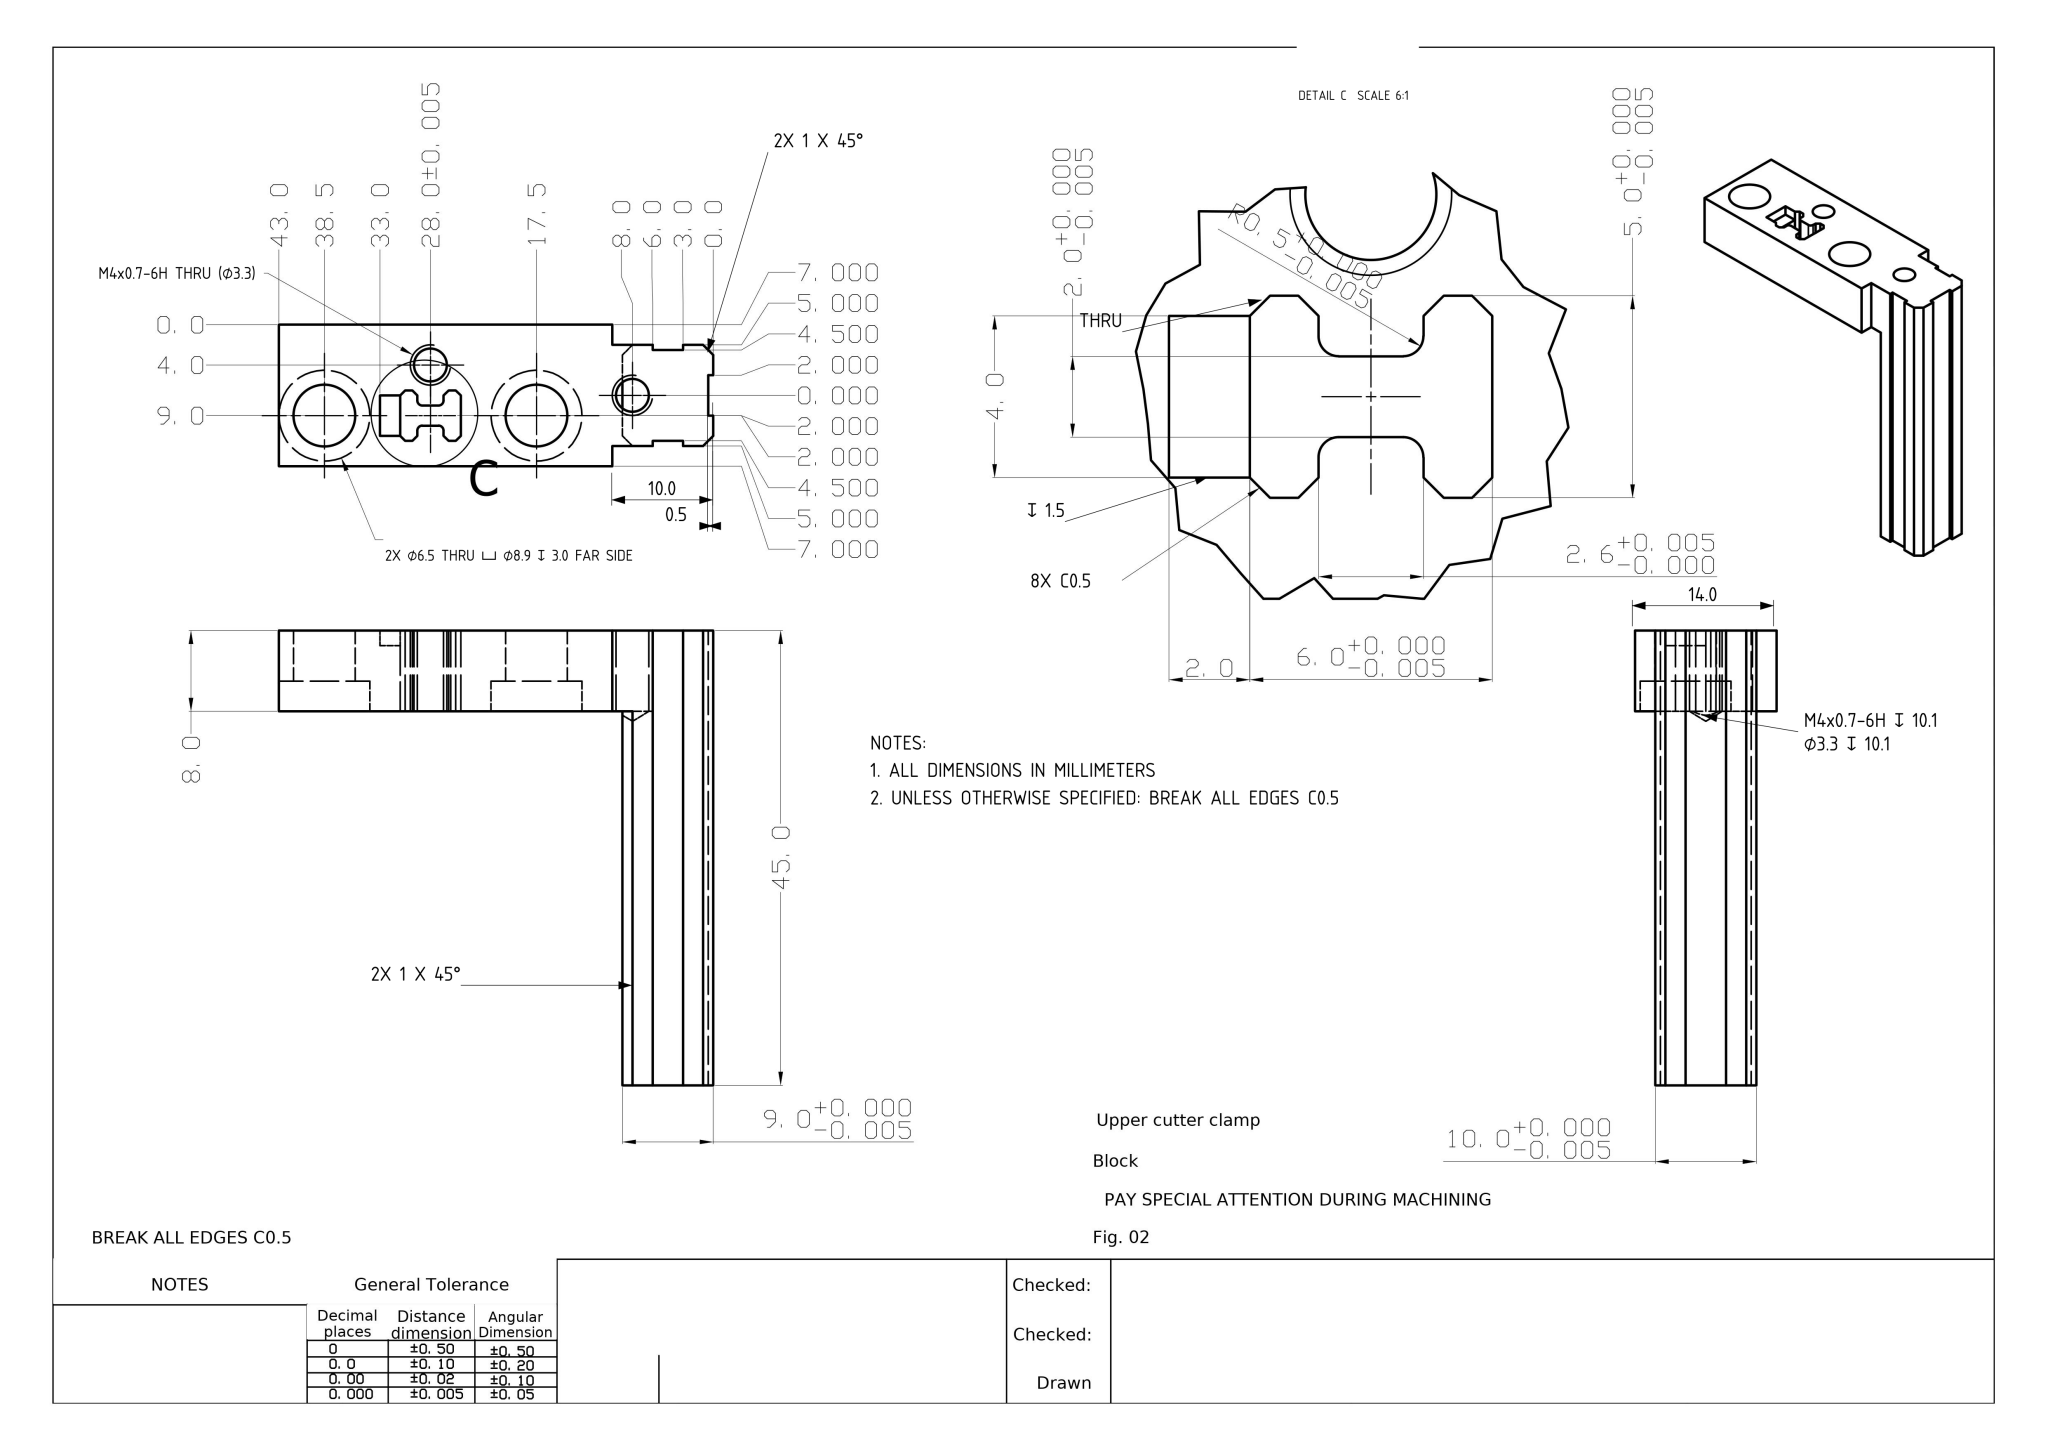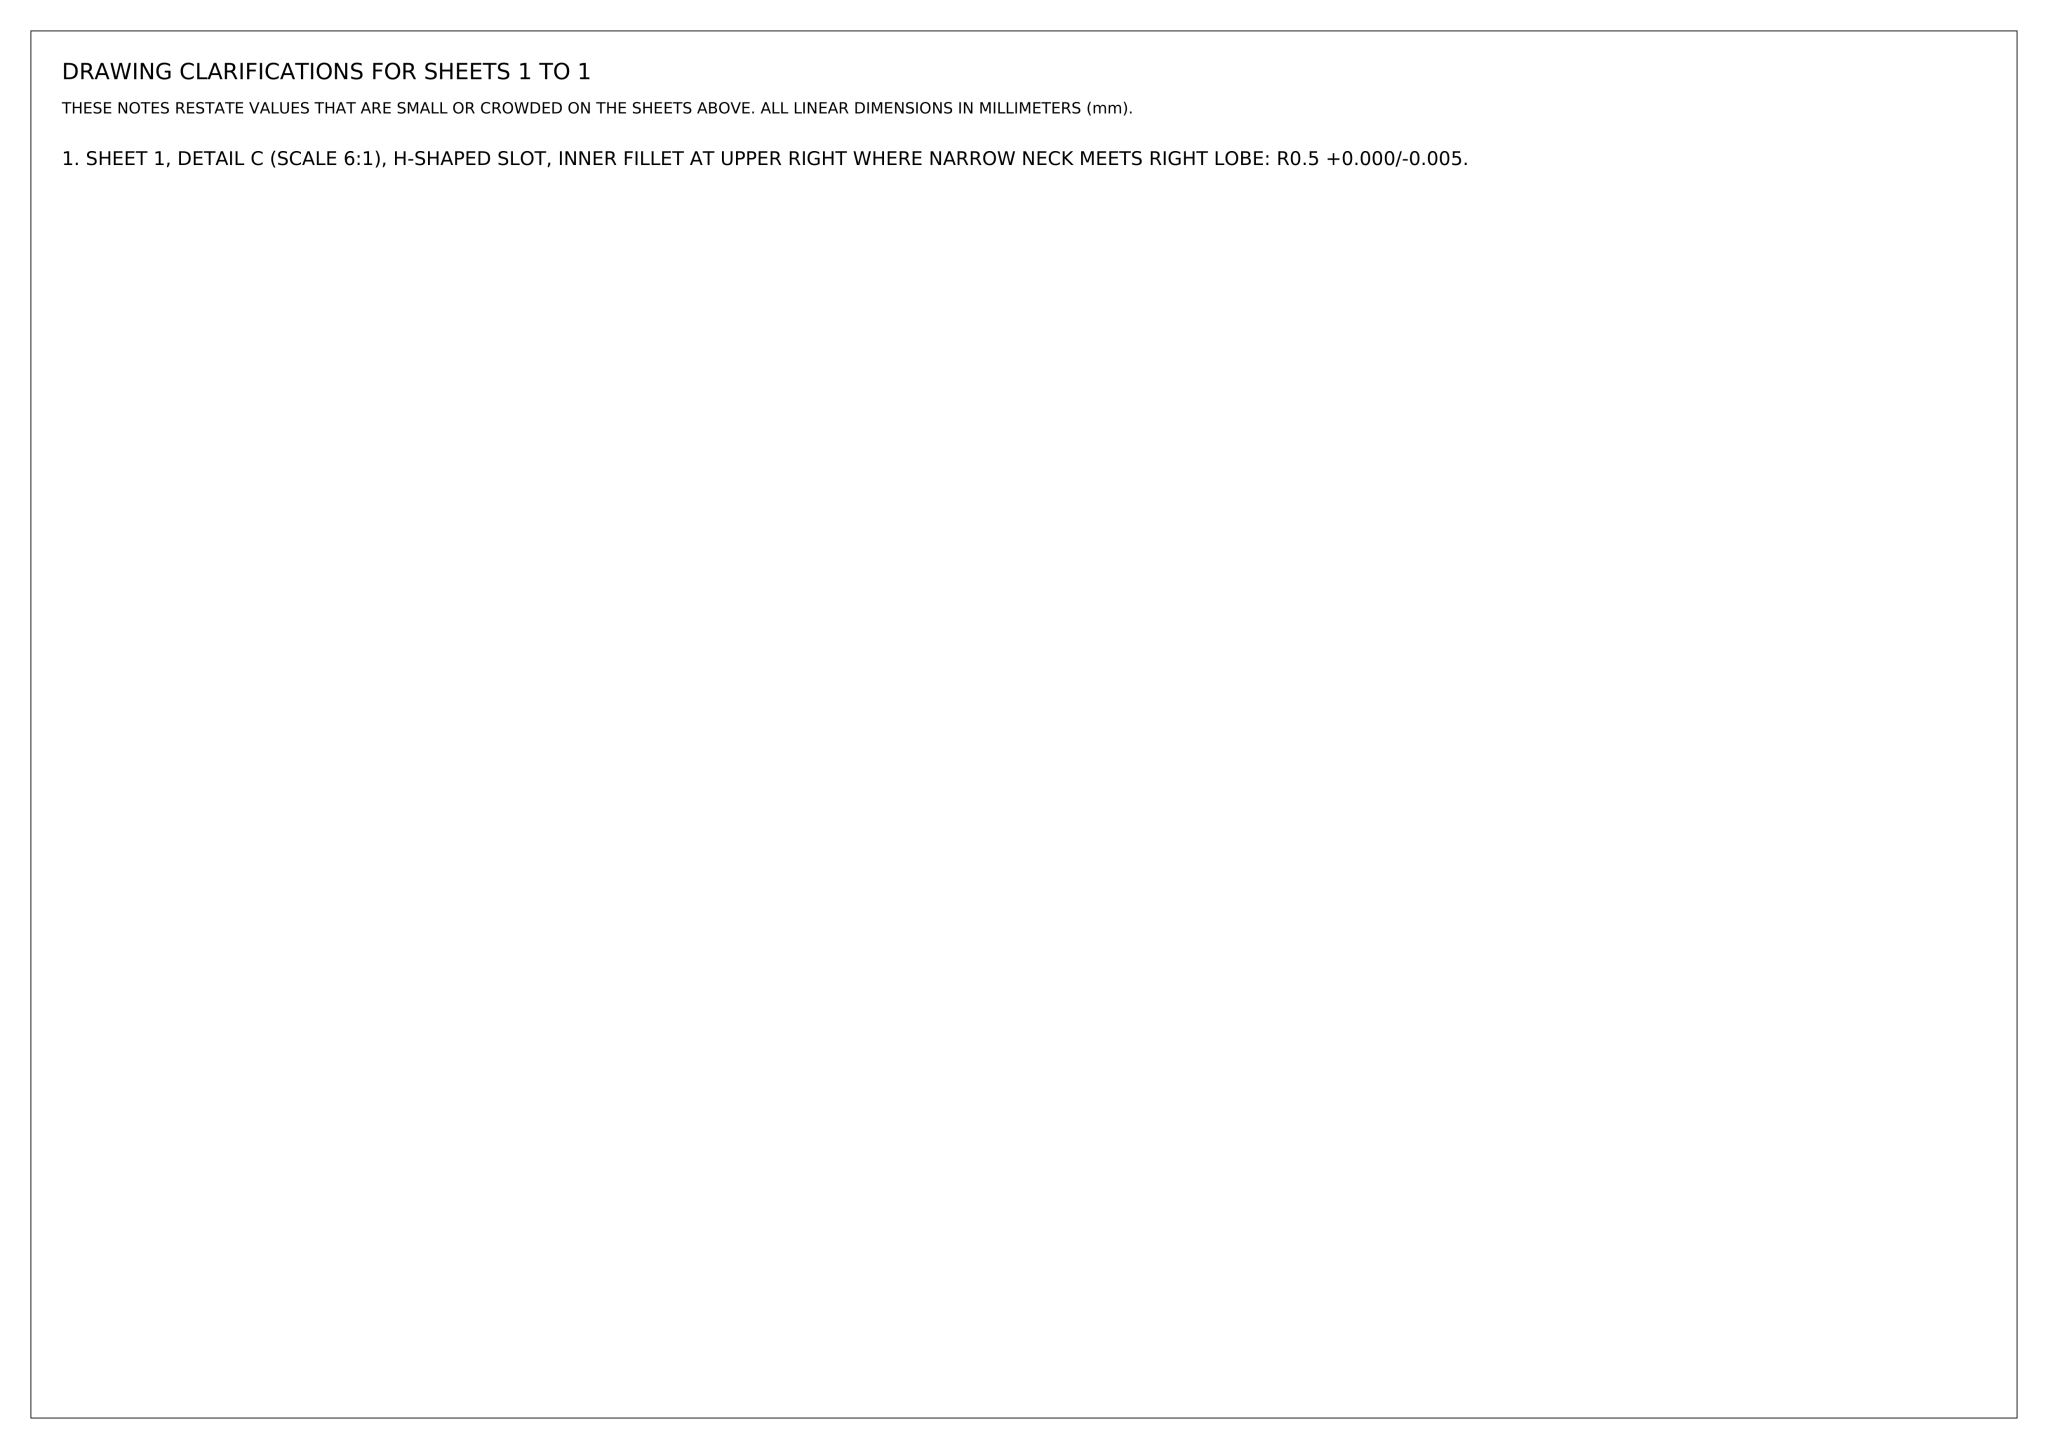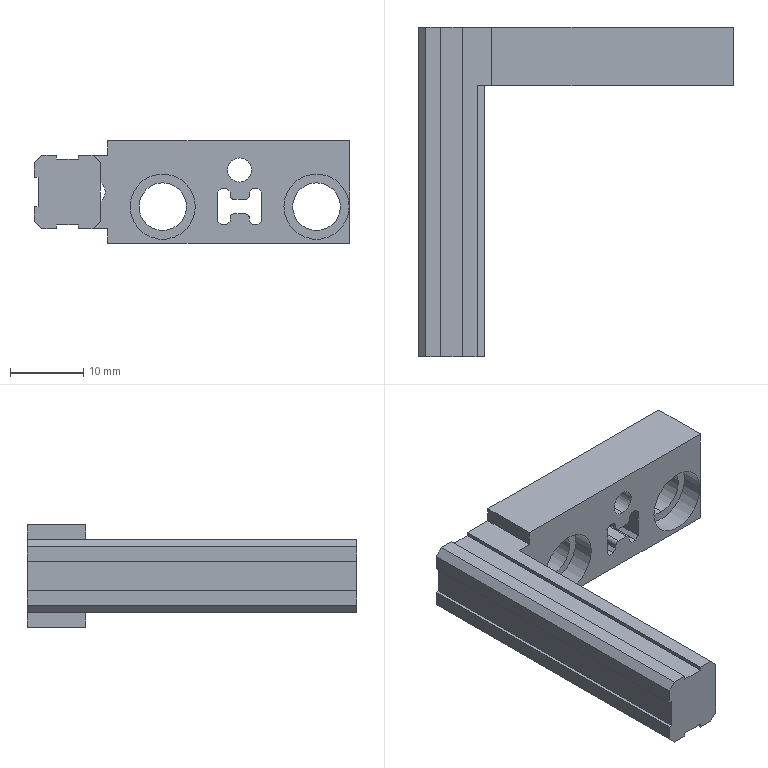Part | NX | mm | 1 solid | 72 faces | box 43 x 45 x 14 mm | volume 6476 mm3 | plane 54 | cylinder 16 | cone 2 | commonest cylinder face diameters 3.3 x4 6.5 x4 8.9 x4 1 x4